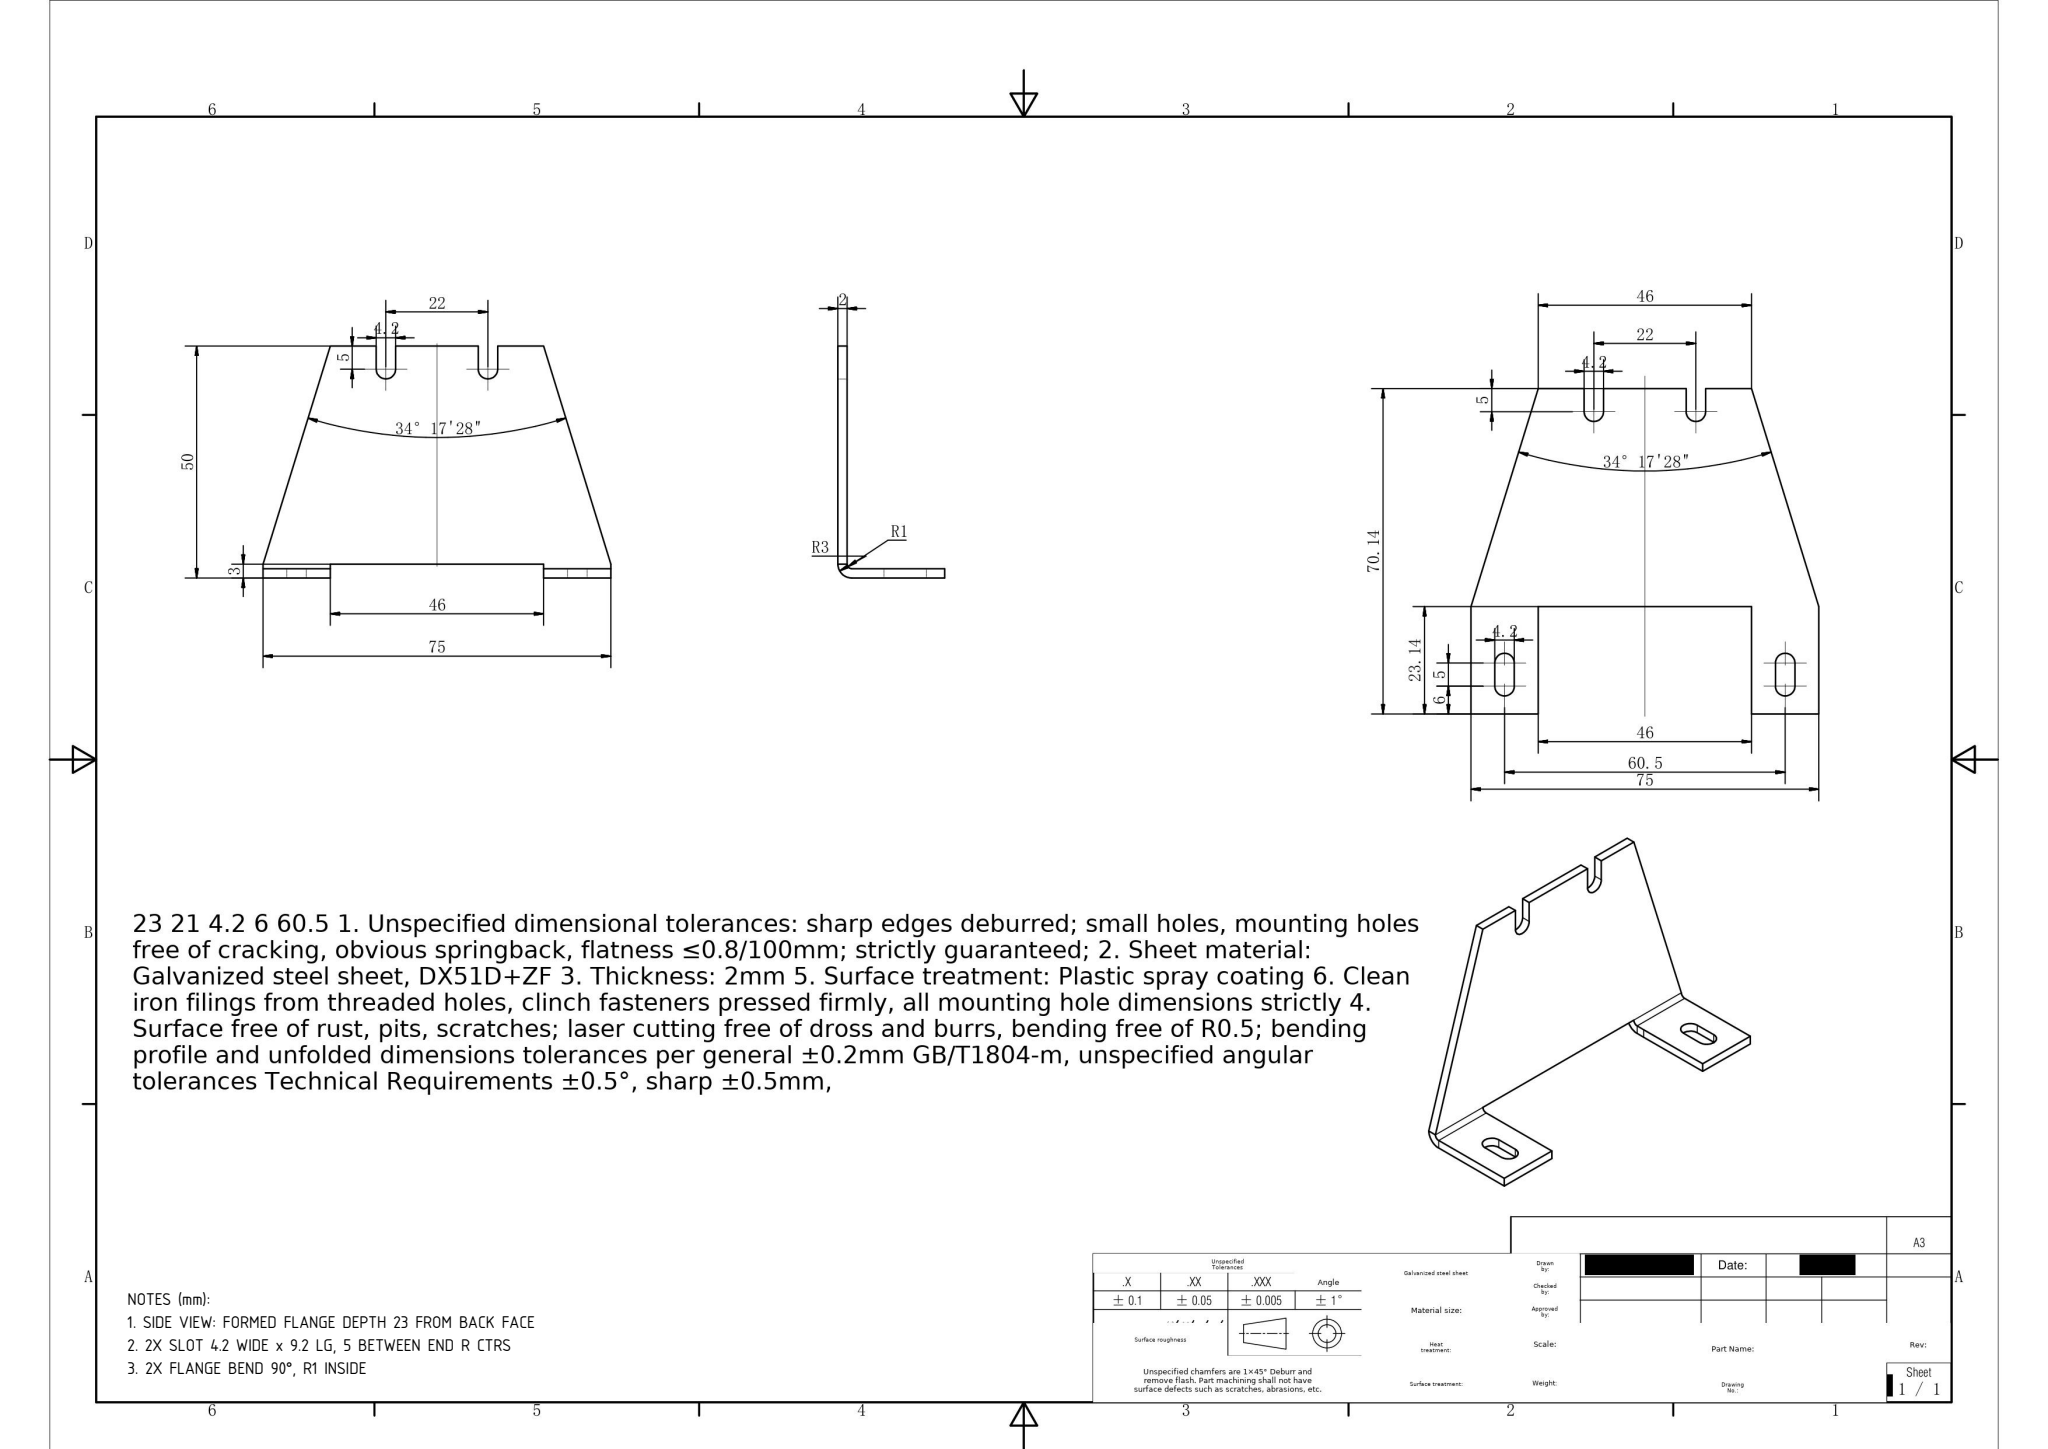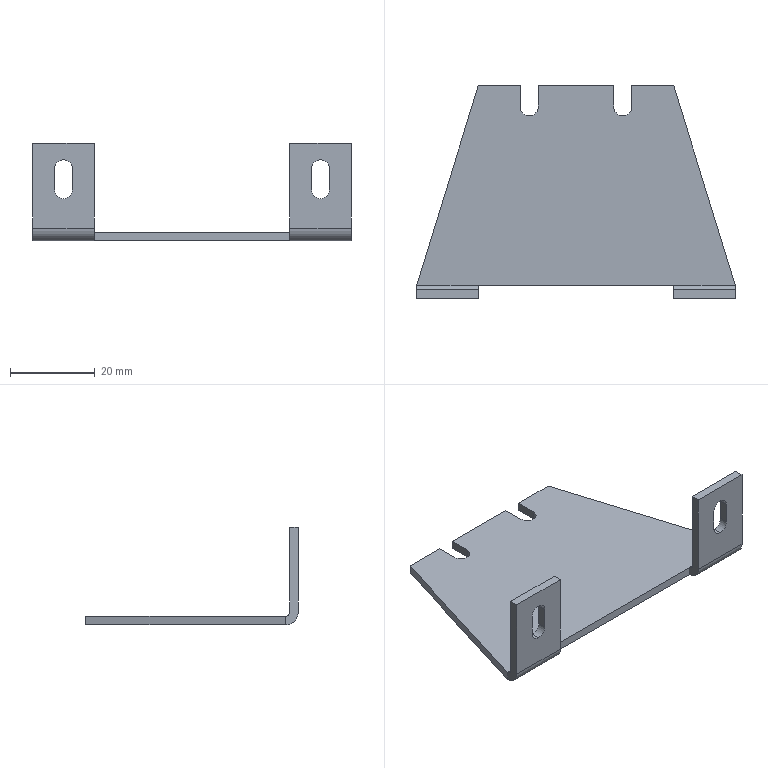Part | SolidWorks | mm | 1 solid | 38 faces | box 75 x 50 x 23 mm | volume 6778 mm3 | plane 26 | cylinder 12 | commonest cylinder face diameters 4.2 x8 2 x2 6 x2
Drawing notes:
SIDE VIEW: FORMED FLANGE DEPTH 23 FROM BACK FACE | from the solid: bbox_xyz z = 23.0; z planes at 0.0, 2.0 and 23.0 give formed leg length 23
2X SLOT 4.2 WIDE x 9.2 LG, 5 BETWEEN END R CTRS | from the solid: Ø4.2 y-axis cyls at z=12.0 and z=17.0 (x=7.25 & 67.75): 5 apart, 5+4.2=9.2 overall
2X FLANGE BEND 90°, R1 INSIDE | from the solid: y-planes 0/2 (flange faces) normal to z-planes 0/2 (web faces) = 90° bend